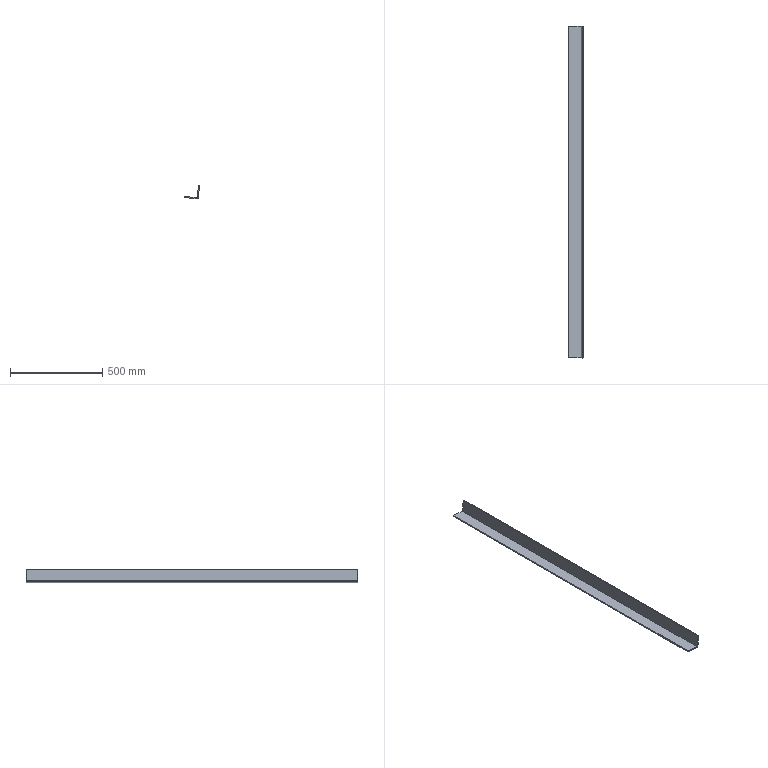Component | NX | UP_RIGHT_FRAME1800_2 | 1 solid | 8 faces | box 82.08 x 1800 x 75.23 mm | volume 1555200 mm3 | plane 8
STEP:
#1=CARTESIAN_POINT('',(0.,0.,0.));
#2=DIRECTION('',(0.,0.,1.));
#3=DIRECTION('',(1.,0.,0.));
#4=AXIS2_PLACEMENT_3D('',#1,#2,#3);
#5=CARTESIAN_POINT('',(1554.12,-7.5,442.548));
#6=VERTEX_POINT('',#5);
#7=CARTESIAN_POINT('',(1479.491,-7.5,449.997));
#8=VERTEX_POINT('',#7);
#9=CARTESIAN_POINT('',(1554.12,-7.5,442.548));
#10=DIRECTION('',(-0.9951,0.,0.09932));
#11=VECTOR('',#10,1.);
#12=LINE('',#9,#11);
#13=CARTESIAN_POINT('',(1554.12,1792.5,442.548));
#14=DIRECTION('',(0.09932,0.,0.9951));
#15=DIRECTION('',(0.9951,0.,-0.09932));
#16=AXIS2_PLACEMENT_3D('',#13,#14,#15);
#17=PLANE('',#16);
#18=CARTESIAN_POINT('',(0.,-1800.));
#19=DIRECTION('',(-1.,0.));
#20=VECTOR('',#19,1.);
#21=LINE('',#18,#20);
#22=(GEOMETRIC_REPRESENTATION_CONTEXT(2)PARAMETRIC_REPRESENTATION_CONTEXT()REPRESENTATION_CONTEXT('',''));
#23=DEFINITIONAL_REPRESENTATION('',(#21),#22);
#24=PCURVE('',#17,#23);
#25=CARTESIAN_POINT('',(1479.491,-7.5,449.997));
#26=DIRECTION('',(0.,1.,0.));
#27=DIRECTION('',(-0.9951,0.,0.09932));
#28=AXIS2_PLACEMENT_3D('',#25,#26,#27);
#29=PLANE('',#28);
#30=CARTESIAN_POINT('',(-75.,-0.));
#31=DIRECTION('',(1.,0.));
#32=VECTOR('',#31,1.);
#33=LINE('',#30,#32);
#34=(GEOMETRIC_REPRESENTATION_CONTEXT(2)PARAMETRIC_REPRESENTATION_CONTEXT()REPRESENTATION_CONTEXT('',''));
#35=DEFINITIONAL_REPRESENTATION('',(#33),#34);
#36=PCURVE('',#29,#35);
#37=SURFACE_CURVE('',#12,(#24,#36),.PCURVE_S1.);
#38=EDGE_CURVE('',#6,#8,#37,.T.);
#39=ORIENTED_EDGE('',*,*,#38,.T.);
#40=CARTESIAN_POINT('',(1479.491,1792.5,449.997));
#41=VERTEX_POINT('',#40);
#42=CARTESIAN_POINT('',(1479.491,1792.5,449.997));
#43=DIRECTION('',(0.,-1.,0.));
#44=VECTOR('',#43,1.);
#45=LINE('',#42,#44);
#46=CARTESIAN_POINT('',(-75.,0.));
#47=DIRECTION('',(0.,-1.));
#48=VECTOR('',#47,1.);
#49=LINE('',#46,#48);
#50=(GEOMETRIC_REPRESENTATION_CONTEXT(2)PARAMETRIC_REPRESENTATION_CONTEXT()REPRESENTATION_CONTEXT('',''));
#51=DEFINITIONAL_REPRESENTATION('',(#49),#50);
#52=PCURVE('',#17,#51);
#53=CARTESIAN_POINT('',(1479.491,1792.5,449.997));
#54=DIRECTION('',(0.9951,0.,-0.09932));
#55=DIRECTION('',(-0.09932,0.,-0.9951));
#56=AXIS2_PLACEMENT_3D('',#53,#54,#55);
#57=PLANE('',#56);
#58=CARTESIAN_POINT('',(0.,0.));
#59=DIRECTION('',(0.,-1.));
#60=VECTOR('',#59,1.);
#61=LINE('',#58,#60);
#62=(GEOMETRIC_REPRESENTATION_CONTEXT(2)PARAMETRIC_REPRESENTATION_CONTEXT()REPRESENTATION_CONTEXT('',''));
#63=DEFINITIONAL_REPRESENTATION('',(#61),#62);
#64=PCURVE('',#57,#63);
#65=SURFACE_CURVE('',#45,(#52,#64),.PCURVE_S1.);
#66=EDGE_CURVE('',#41,#8,#65,.T.);
#67=ORIENTED_EDGE('',*,*,#66,.F.);
#68=CARTESIAN_POINT('',(1554.12,1792.5,442.548));
#69=VERTEX_POINT('',#68);
#70=CARTESIAN_POINT('',(1554.12,1792.5,442.548));
#71=DIRECTION('',(-0.9951,0.,0.09932));
#72=VECTOR('',#71,1.);
#73=LINE('',#70,#72);
#74=CARTESIAN_POINT('',(0.,0.));
#75=DIRECTION('',(-1.,0.));
#76=VECTOR('',#75,1.);
#77=LINE('',#74,#76);
#78=(GEOMETRIC_REPRESENTATION_CONTEXT(2)PARAMETRIC_REPRESENTATION_CONTEXT()REPRESENTATION_CONTEXT('',''));
#79=DEFINITIONAL_REPRESENTATION('',(#77),#78);
#80=PCURVE('',#17,#79);
#81=CARTESIAN_POINT('',(1479.491,1792.5,449.997));
#82=DIRECTION('',(0.,1.,0.));
#83=DIRECTION('',(-0.9951,0.,0.09932));
#84=AXIS2_PLACEMENT_3D('',#81,#82,#83);
#85=PLANE('',#84);
#86=CARTESIAN_POINT('',(-75.,-0.));
#87=DIRECTION('',(1.,0.));
#88=VECTOR('',#87,1.);
#89=LINE('',#86,#88);
#90=(GEOMETRIC_REPRESENTATION_CONTEXT(2)PARAMETRIC_REPRESENTATION_CONTEXT()REPRESENTATION_CONTEXT('',''));
#91=DEFINITIONAL_REPRESENTATION('',(#89),#90);
#92=PCURVE('',#85,#91);
#93=SURFACE_CURVE('',#73,(#80,#92),.PCURVE_S1.);
#94=EDGE_CURVE('',#69,#41,#93,.T.);
#95=ORIENTED_EDGE('',*,*,#94,.F.);
#96=CARTESIAN_POINT('',(1554.12,1792.5,442.548));
#97=DIRECTION('',(0.,-1.,0.));
#98=VECTOR('',#97,1.);
#99=LINE('',#96,#98);
#100=CARTESIAN_POINT('',(0.,0.));
#101=DIRECTION('',(0.,-1.));
#102=VECTOR('',#101,1.);
#103=LINE('',#100,#102);
#104=(GEOMETRIC_REPRESENTATION_CONTEXT(2)PARAMETRIC_REPRESENTATION_CONTEXT()REPRESENTATION_CONTEXT('',''));
#105=DEFINITIONAL_REPRESENTATION('',(#103),#104);
#106=PCURVE('',#17,#105);
#107=CARTESIAN_POINT('',(1561.569,1792.5,517.177));
#108=DIRECTION('',(-0.9951,0.,0.09932));
#109=DIRECTION('',(0.09932,0.,0.9951));
#110=AXIS2_PLACEMENT_3D('',#107,#108,#109);
#111=PLANE('',#110);
#112=CARTESIAN_POINT('',(-75.,0.));
#113=DIRECTION('',(0.,-1.));
#114=VECTOR('',#113,1.);
#115=LINE('',#112,#114);
#116=(GEOMETRIC_REPRESENTATION_CONTEXT(2)PARAMETRIC_REPRESENTATION_CONTEXT()REPRESENTATION_CONTEXT('',''));
#117=DEFINITIONAL_REPRESENTATION('',(#115),#116);
#118=PCURVE('',#111,#117);
#119=SURFACE_CURVE('',#99,(#106,#118),.PCURVE_S1.);
#120=EDGE_CURVE('',#69,#6,#119,.T.);
#121=ORIENTED_EDGE('',*,*,#120,.T.);
#122=EDGE_LOOP('',(#39,#67,#95,#121));
#123=FACE_BOUND('',#122,.T.);
#124=ADVANCED_FACE('',(#123),#17,.F.);
#125=CARTESIAN_POINT('',(1480.087,-7.5,455.967));
#126=VERTEX_POINT('',#125);
#127=CARTESIAN_POINT('',(1479.491,-7.5,449.997));
#128=DIRECTION('',(0.09932,0.,0.9951));
#129=VECTOR('',#128,1.);
#130=LINE('',#127,#129);
#131=CARTESIAN_POINT('',(0.,-1800.));
#132=DIRECTION('',(-1.,0.));
#133=VECTOR('',#132,1.);
#134=LINE('',#131,#133);
#135=(GEOMETRIC_REPRESENTATION_CONTEXT(2)PARAMETRIC_REPRESENTATION_CONTEXT()REPRESENTATION_CONTEXT('',''));
#136=DEFINITIONAL_REPRESENTATION('',(#134),#135);
#137=PCURVE('',#57,#136);
#138=CARTESIAN_POINT('',(0.,0.));
#139=DIRECTION('',(0.,1.));
#140=VECTOR('',#139,1.);
#141=LINE('',#138,#140);
#142=(GEOMETRIC_REPRESENTATION_CONTEXT(2)PARAMETRIC_REPRESENTATION_CONTEXT()REPRESENTATION_CONTEXT('',''));
#143=DEFINITIONAL_REPRESENTATION('',(#141),#142);
#144=PCURVE('',#29,#143);
#145=SURFACE_CURVE('',#130,(#137,#144),.PCURVE_S1.);
#146=EDGE_CURVE('',#8,#126,#145,.T.);
#147=ORIENTED_EDGE('',*,*,#146,.T.);
#148=CARTESIAN_POINT('',(1480.087,1792.5,455.967));
#149=VERTEX_POINT('',#148);
#150=CARTESIAN_POINT('',(1480.087,1792.5,455.967));
#151=DIRECTION('',(0.,-1.,0.));
#152=VECTOR('',#151,1.);
#153=LINE('',#150,#152);
#154=CARTESIAN_POINT('',(-6.,0.));
#155=DIRECTION('',(0.,-1.));
#156=VECTOR('',#155,1.);
#157=LINE('',#154,#156);
#158=(GEOMETRIC_REPRESENTATION_CONTEXT(2)PARAMETRIC_REPRESENTATION_CONTEXT()REPRESENTATION_CONTEXT('',''));
#159=DEFINITIONAL_REPRESENTATION('',(#157),#158);
#160=PCURVE('',#57,#159);
#161=CARTESIAN_POINT('',(1480.087,1792.5,455.967));
#162=DIRECTION('',(-0.09932,0.,-0.9951));
#163=DIRECTION('',(-0.9951,0.,0.09932));
#164=AXIS2_PLACEMENT_3D('',#161,#162,#163);
#165=PLANE('',#164);
#166=CARTESIAN_POINT('',(0.,0.));
#167=DIRECTION('',(0.,-1.));
#168=VECTOR('',#167,1.);
#169=LINE('',#166,#168);
#170=(GEOMETRIC_REPRESENTATION_CONTEXT(2)PARAMETRIC_REPRESENTATION_CONTEXT()REPRESENTATION_CONTEXT('',''));
#171=DEFINITIONAL_REPRESENTATION('',(#169),#170);
#172=PCURVE('',#165,#171);
#173=SURFACE_CURVE('',#153,(#160,#172),.PCURVE_S1.);
#174=EDGE_CURVE('',#149,#126,#173,.T.);
#175=ORIENTED_EDGE('',*,*,#174,.F.);
#176=CARTESIAN_POINT('',(1479.491,1792.5,449.997));
#177=DIRECTION('',(0.09932,0.,0.9951));
#178=VECTOR('',#177,1.);
#179=LINE('',#176,#178);
#180=CARTESIAN_POINT('',(0.,0.));
#181=DIRECTION('',(-1.,0.));
#182=VECTOR('',#181,1.);
#183=LINE('',#180,#182);
#184=(GEOMETRIC_REPRESENTATION_CONTEXT(2)PARAMETRIC_REPRESENTATION_CONTEXT()REPRESENTATION_CONTEXT('',''));
#185=DEFINITIONAL_REPRESENTATION('',(#183),#184);
#186=PCURVE('',#57,#185);
#187=CARTESIAN_POINT('',(0.,0.));
#188=DIRECTION('',(0.,1.));
#189=VECTOR('',#188,1.);
#190=LINE('',#187,#189);
#191=(GEOMETRIC_REPRESENTATION_CONTEXT(2)PARAMETRIC_REPRESENTATION_CONTEXT()REPRESENTATION_CONTEXT('',''));
#192=DEFINITIONAL_REPRESENTATION('',(#190),#191);
#193=PCURVE('',#85,#192);
#194=SURFACE_CURVE('',#179,(#186,#193),.PCURVE_S1.);
#195=EDGE_CURVE('',#41,#149,#194,.T.);
#196=ORIENTED_EDGE('',*,*,#195,.F.);
#197=ORIENTED_EDGE('',*,*,#66,.T.);
#198=EDGE_LOOP('',(#147,#175,#196,#197));
#199=FACE_BOUND('',#198,.T.);
#200=ADVANCED_FACE('',(#199),#57,.F.);
#201=CARTESIAN_POINT('',(1548.746,-7.5,449.114));
#202=VERTEX_POINT('',#201);
#203=CARTESIAN_POINT('',(1480.087,-7.5,455.967));
#204=DIRECTION('',(0.9951,0.,-0.09932));
#205=VECTOR('',#204,1.);
#206=LINE('',#203,#205);
#207=CARTESIAN_POINT('',(0.,-1800.));
#208=DIRECTION('',(-1.,0.));
#209=VECTOR('',#208,1.);
#210=LINE('',#207,#209);
#211=(GEOMETRIC_REPRESENTATION_CONTEXT(2)PARAMETRIC_REPRESENTATION_CONTEXT()REPRESENTATION_CONTEXT('',''));
#212=DEFINITIONAL_REPRESENTATION('',(#210),#211);
#213=PCURVE('',#165,#212);
#214=CARTESIAN_POINT('',(0.,6.));
#215=DIRECTION('',(-1.,-0.));
#216=VECTOR('',#215,1.);
#217=LINE('',#214,#216);
#218=(GEOMETRIC_REPRESENTATION_CONTEXT(2)PARAMETRIC_REPRESENTATION_CONTEXT()REPRESENTATION_CONTEXT('',''));
#219=DEFINITIONAL_REPRESENTATION('',(#217),#218);
#220=PCURVE('',#29,#219);
#221=SURFACE_CURVE('',#206,(#213,#220),.PCURVE_S1.);
#222=EDGE_CURVE('',#126,#202,#221,.T.);
#223=ORIENTED_EDGE('',*,*,#222,.T.);
#224=CARTESIAN_POINT('',(1548.746,1792.5,449.114));
#225=VERTEX_POINT('',#224);
#226=CARTESIAN_POINT('',(1548.746,1792.5,449.114));
#227=DIRECTION('',(0.,-1.,0.));
#228=VECTOR('',#227,1.);
#229=LINE('',#226,#228);
#230=CARTESIAN_POINT('',(-69.,0.));
#231=DIRECTION('',(0.,-1.));
#232=VECTOR('',#231,1.);
#233=LINE('',#230,#232);
#234=(GEOMETRIC_REPRESENTATION_CONTEXT(2)PARAMETRIC_REPRESENTATION_CONTEXT()REPRESENTATION_CONTEXT('',''));
#235=DEFINITIONAL_REPRESENTATION('',(#233),#234);
#236=PCURVE('',#165,#235);
#237=CARTESIAN_POINT('',(1548.746,1792.5,449.114));
#238=DIRECTION('',(0.9951,0.,-0.09932));
#239=DIRECTION('',(-0.09932,0.,-0.9951));
#240=AXIS2_PLACEMENT_3D('',#237,#238,#239);
#241=PLANE('',#240);
#242=CARTESIAN_POINT('',(0.,0.));
#243=DIRECTION('',(0.,-1.));
#244=VECTOR('',#243,1.);
#245=LINE('',#242,#244);
#246=(GEOMETRIC_REPRESENTATION_CONTEXT(2)PARAMETRIC_REPRESENTATION_CONTEXT()REPRESENTATION_CONTEXT('',''));
#247=DEFINITIONAL_REPRESENTATION('',(#245),#246);
#248=PCURVE('',#241,#247);
#249=SURFACE_CURVE('',#229,(#236,#248),.PCURVE_S1.);
#250=EDGE_CURVE('',#225,#202,#249,.T.);
#251=ORIENTED_EDGE('',*,*,#250,.F.);
#252=CARTESIAN_POINT('',(1480.087,1792.5,455.967));
#253=DIRECTION('',(0.9951,0.,-0.09932));
#254=VECTOR('',#253,1.);
#255=LINE('',#252,#254);
#256=CARTESIAN_POINT('',(0.,0.));
#257=DIRECTION('',(-1.,0.));
#258=VECTOR('',#257,1.);
#259=LINE('',#256,#258);
#260=(GEOMETRIC_REPRESENTATION_CONTEXT(2)PARAMETRIC_REPRESENTATION_CONTEXT()REPRESENTATION_CONTEXT('',''));
#261=DEFINITIONAL_REPRESENTATION('',(#259),#260);
#262=PCURVE('',#165,#261);
#263=CARTESIAN_POINT('',(0.,6.));
#264=DIRECTION('',(-1.,-0.));
#265=VECTOR('',#264,1.);
#266=LINE('',#263,#265);
#267=(GEOMETRIC_REPRESENTATION_CONTEXT(2)PARAMETRIC_REPRESENTATION_CONTEXT()REPRESENTATION_CONTEXT('',''));
#268=DEFINITIONAL_REPRESENTATION('',(#266),#267);
#269=PCURVE('',#85,#268);
#270=SURFACE_CURVE('',#255,(#262,#269),.PCURVE_S1.);
#271=EDGE_CURVE('',#149,#225,#270,.T.);
#272=ORIENTED_EDGE('',*,*,#271,.F.);
#273=ORIENTED_EDGE('',*,*,#174,.T.);
#274=EDGE_LOOP('',(#223,#251,#272,#273));
#275=FACE_BOUND('',#274,.T.);
#276=ADVANCED_FACE('',(#275),#165,.F.);
#277=CARTESIAN_POINT('',(1555.599,-7.5,517.773));
#278=VERTEX_POINT('',#277);
#279=CARTESIAN_POINT('',(1548.746,-7.5,449.114));
#280=DIRECTION('',(0.09932,0.,0.9951));
#281=VECTOR('',#280,1.);
#282=LINE('',#279,#281);
#283=CARTESIAN_POINT('',(0.,-1800.));
#284=DIRECTION('',(-1.,0.));
#285=VECTOR('',#284,1.);
#286=LINE('',#283,#285);
#287=(GEOMETRIC_REPRESENTATION_CONTEXT(2)PARAMETRIC_REPRESENTATION_CONTEXT()REPRESENTATION_CONTEXT('',''));
#288=DEFINITIONAL_REPRESENTATION('',(#286),#287);
#289=PCURVE('',#241,#288);
#290=CARTESIAN_POINT('',(-69.,6.));
#291=DIRECTION('',(0.,1.));
#292=VECTOR('',#291,1.);
#293=LINE('',#290,#292);
#294=(GEOMETRIC_REPRESENTATION_CONTEXT(2)PARAMETRIC_REPRESENTATION_CONTEXT()REPRESENTATION_CONTEXT('',''));
#295=DEFINITIONAL_REPRESENTATION('',(#293),#294);
#296=PCURVE('',#29,#295);
#297=SURFACE_CURVE('',#282,(#289,#296),.PCURVE_S1.);
#298=EDGE_CURVE('',#202,#278,#297,.T.);
#299=ORIENTED_EDGE('',*,*,#298,.T.);
#300=CARTESIAN_POINT('',(1555.599,1792.5,517.773));
#301=VERTEX_POINT('',#300);
#302=CARTESIAN_POINT('',(1555.599,1792.5,517.773));
#303=DIRECTION('',(0.,-1.,0.));
#304=VECTOR('',#303,1.);
#305=LINE('',#302,#304);
#306=CARTESIAN_POINT('',(-69.,0.));
#307=DIRECTION('',(0.,-1.));
#308=VECTOR('',#307,1.);
#309=LINE('',#306,#308);
#310=(GEOMETRIC_REPRESENTATION_CONTEXT(2)PARAMETRIC_REPRESENTATION_CONTEXT()REPRESENTATION_CONTEXT('',''));
#311=DEFINITIONAL_REPRESENTATION('',(#309),#310);
#312=PCURVE('',#241,#311);
#313=CARTESIAN_POINT('',(1555.599,1792.5,517.773));
#314=DIRECTION('',(-0.09932,0.,-0.9951));
#315=DIRECTION('',(-0.9951,0.,0.09932));
#316=AXIS2_PLACEMENT_3D('',#313,#314,#315);
#317=PLANE('',#316);
#318=CARTESIAN_POINT('',(0.,0.));
#319=DIRECTION('',(0.,-1.));
#320=VECTOR('',#319,1.);
#321=LINE('',#318,#320);
#322=(GEOMETRIC_REPRESENTATION_CONTEXT(2)PARAMETRIC_REPRESENTATION_CONTEXT()REPRESENTATION_CONTEXT('',''));
#323=DEFINITIONAL_REPRESENTATION('',(#321),#322);
#324=PCURVE('',#317,#323);
#325=SURFACE_CURVE('',#305,(#312,#324),.PCURVE_S1.);
#326=EDGE_CURVE('',#301,#278,#325,.T.);
#327=ORIENTED_EDGE('',*,*,#326,.F.);
#328=CARTESIAN_POINT('',(1548.746,1792.5,449.114));
#329=DIRECTION('',(0.09932,0.,0.9951));
#330=VECTOR('',#329,1.);
#331=LINE('',#328,#330);
#332=CARTESIAN_POINT('',(0.,0.));
#333=DIRECTION('',(-1.,0.));
#334=VECTOR('',#333,1.);
#335=LINE('',#332,#334);
#336=(GEOMETRIC_REPRESENTATION_CONTEXT(2)PARAMETRIC_REPRESENTATION_CONTEXT()REPRESENTATION_CONTEXT('',''));
#337=DEFINITIONAL_REPRESENTATION('',(#335),#336);
#338=PCURVE('',#241,#337);
#339=CARTESIAN_POINT('',(-69.,6.));
#340=DIRECTION('',(0.,1.));
#341=VECTOR('',#340,1.);
#342=LINE('',#339,#341);
#343=(GEOMETRIC_REPRESENTATION_CONTEXT(2)PARAMETRIC_REPRESENTATION_CONTEXT()REPRESENTATION_CONTEXT('',''));
#344=DEFINITIONAL_REPRESENTATION('',(#342),#343);
#345=PCURVE('',#85,#344);
#346=SURFACE_CURVE('',#331,(#338,#345),.PCURVE_S1.);
#347=EDGE_CURVE('',#225,#301,#346,.T.);
#348=ORIENTED_EDGE('',*,*,#347,.F.);
#349=ORIENTED_EDGE('',*,*,#250,.T.);
#350=EDGE_LOOP('',(#299,#327,#348,#349));
#351=FACE_BOUND('',#350,.T.);
#352=ADVANCED_FACE('',(#351),#241,.F.);
#353=CARTESIAN_POINT('',(1561.569,-7.5,517.177));
#354=VERTEX_POINT('',#353);
#355=CARTESIAN_POINT('',(1555.599,-7.5,517.773));
#356=DIRECTION('',(0.9951,0.,-0.09932));
#357=VECTOR('',#356,1.);
#358=LINE('',#355,#357);
#359=CARTESIAN_POINT('',(0.,-1800.));
#360=DIRECTION('',(-1.,0.));
#361=VECTOR('',#360,1.);
#362=LINE('',#359,#361);
#363=(GEOMETRIC_REPRESENTATION_CONTEXT(2)PARAMETRIC_REPRESENTATION_CONTEXT()REPRESENTATION_CONTEXT('',''));
#364=DEFINITIONAL_REPRESENTATION('',(#362),#363);
#365=PCURVE('',#317,#364);
#366=CARTESIAN_POINT('',(-69.,75.));
#367=DIRECTION('',(-1.,0.));
#368=VECTOR('',#367,1.);
#369=LINE('',#366,#368);
#370=(GEOMETRIC_REPRESENTATION_CONTEXT(2)PARAMETRIC_REPRESENTATION_CONTEXT()REPRESENTATION_CONTEXT('',''));
#371=DEFINITIONAL_REPRESENTATION('',(#369),#370);
#372=PCURVE('',#29,#371);
#373=SURFACE_CURVE('',#358,(#365,#372),.PCURVE_S1.);
#374=EDGE_CURVE('',#278,#354,#373,.T.);
#375=ORIENTED_EDGE('',*,*,#374,.T.);
#376=CARTESIAN_POINT('',(1561.569,1792.5,517.177));
#377=VERTEX_POINT('',#376);
#378=CARTESIAN_POINT('',(1561.569,1792.5,517.177));
#379=DIRECTION('',(0.,-1.,0.));
#380=VECTOR('',#379,1.);
#381=LINE('',#378,#380);
#382=CARTESIAN_POINT('',(-6.,0.));
#383=DIRECTION('',(0.,-1.));
#384=VECTOR('',#383,1.);
#385=LINE('',#382,#384);
#386=(GEOMETRIC_REPRESENTATION_CONTEXT(2)PARAMETRIC_REPRESENTATION_CONTEXT()REPRESENTATION_CONTEXT('',''));
#387=DEFINITIONAL_REPRESENTATION('',(#385),#386);
#388=PCURVE('',#317,#387);
#389=CARTESIAN_POINT('',(0.,0.));
#390=DIRECTION('',(0.,-1.));
#391=VECTOR('',#390,1.);
#392=LINE('',#389,#391);
#393=(GEOMETRIC_REPRESENTATION_CONTEXT(2)PARAMETRIC_REPRESENTATION_CONTEXT()REPRESENTATION_CONTEXT('',''));
#394=DEFINITIONAL_REPRESENTATION('',(#392),#393);
#395=PCURVE('',#111,#394);
#396=SURFACE_CURVE('',#381,(#388,#395),.PCURVE_S1.);
#397=EDGE_CURVE('',#377,#354,#396,.T.);
#398=ORIENTED_EDGE('',*,*,#397,.F.);
#399=CARTESIAN_POINT('',(1555.599,1792.5,517.773));
#400=DIRECTION('',(0.9951,0.,-0.09932));
#401=VECTOR('',#400,1.);
#402=LINE('',#399,#401);
#403=CARTESIAN_POINT('',(0.,0.));
#404=DIRECTION('',(-1.,0.));
#405=VECTOR('',#404,1.);
#406=LINE('',#403,#405);
#407=(GEOMETRIC_REPRESENTATION_CONTEXT(2)PARAMETRIC_REPRESENTATION_CONTEXT()REPRESENTATION_CONTEXT('',''));
#408=DEFINITIONAL_REPRESENTATION('',(#406),#407);
#409=PCURVE('',#317,#408);
#410=CARTESIAN_POINT('',(-69.,75.));
#411=DIRECTION('',(-1.,0.));
#412=VECTOR('',#411,1.);
#413=LINE('',#410,#412);
#414=(GEOMETRIC_REPRESENTATION_CONTEXT(2)PARAMETRIC_REPRESENTATION_CONTEXT()REPRESENTATION_CONTEXT('',''));
#415=DEFINITIONAL_REPRESENTATION('',(#413),#414);
#416=PCURVE('',#85,#415);
#417=SURFACE_CURVE('',#402,(#409,#416),.PCURVE_S1.);
#418=EDGE_CURVE('',#301,#377,#417,.T.);
#419=ORIENTED_EDGE('',*,*,#418,.F.);
#420=ORIENTED_EDGE('',*,*,#326,.T.);
#421=EDGE_LOOP('',(#375,#398,#419,#420));
#422=FACE_BOUND('',#421,.T.);
#423=ADVANCED_FACE('',(#422),#317,.F.);
#424=CARTESIAN_POINT('',(1561.569,-7.5,517.177));
#425=DIRECTION('',(-0.09932,0.,-0.9951));
#426=VECTOR('',#425,1.);
#427=LINE('',#424,#426);
#428=CARTESIAN_POINT('',(0.,-1800.));
#429=DIRECTION('',(-1.,0.));
#430=VECTOR('',#429,1.);
#431=LINE('',#428,#430);
#432=(GEOMETRIC_REPRESENTATION_CONTEXT(2)PARAMETRIC_REPRESENTATION_CONTEXT()REPRESENTATION_CONTEXT('',''));
#433=DEFINITIONAL_REPRESENTATION('',(#431),#432);
#434=PCURVE('',#111,#433);
#435=CARTESIAN_POINT('',(-75.,75.));
#436=DIRECTION('',(0.,-1.));
#437=VECTOR('',#436,1.);
#438=LINE('',#435,#437);
#439=(GEOMETRIC_REPRESENTATION_CONTEXT(2)PARAMETRIC_REPRESENTATION_CONTEXT()REPRESENTATION_CONTEXT('',''));
#440=DEFINITIONAL_REPRESENTATION('',(#438),#439);
#441=PCURVE('',#29,#440);
#442=SURFACE_CURVE('',#427,(#434,#441),.PCURVE_S1.);
#443=EDGE_CURVE('',#354,#6,#442,.T.);
#444=ORIENTED_EDGE('',*,*,#443,.T.);
#445=ORIENTED_EDGE('',*,*,#120,.F.);
#446=CARTESIAN_POINT('',(1561.569,1792.5,517.177));
#447=DIRECTION('',(-0.09932,0.,-0.9951));
#448=VECTOR('',#447,1.);
#449=LINE('',#446,#448);
#450=CARTESIAN_POINT('',(0.,0.));
#451=DIRECTION('',(-1.,0.));
#452=VECTOR('',#451,1.);
#453=LINE('',#450,#452);
#454=(GEOMETRIC_REPRESENTATION_CONTEXT(2)PARAMETRIC_REPRESENTATION_CONTEXT()REPRESENTATION_CONTEXT('',''));
#455=DEFINITIONAL_REPRESENTATION('',(#453),#454);
#456=PCURVE('',#111,#455);
#457=CARTESIAN_POINT('',(-75.,75.));
#458=DIRECTION('',(0.,-1.));
#459=VECTOR('',#458,1.);
#460=LINE('',#457,#459);
#461=(GEOMETRIC_REPRESENTATION_CONTEXT(2)PARAMETRIC_REPRESENTATION_CONTEXT()REPRESENTATION_CONTEXT('',''));
#462=DEFINITIONAL_REPRESENTATION('',(#460),#461);
#463=PCURVE('',#85,#462);
#464=SURFACE_CURVE('',#449,(#456,#463),.PCURVE_S1.);
#465=EDGE_CURVE('',#377,#69,#464,.T.);
#466=ORIENTED_EDGE('',*,*,#465,.F.);
#467=ORIENTED_EDGE('',*,*,#397,.T.);
#468=EDGE_LOOP('',(#444,#445,#466,#467));
#469=FACE_BOUND('',#468,.T.);
#470=ADVANCED_FACE('',(#469),#111,.F.);
#471=ORIENTED_EDGE('',*,*,#94,.T.);
#472=ORIENTED_EDGE('',*,*,#195,.T.);
#473=ORIENTED_EDGE('',*,*,#271,.T.);
#474=ORIENTED_EDGE('',*,*,#347,.T.);
#475=ORIENTED_EDGE('',*,*,#418,.T.);
#476=ORIENTED_EDGE('',*,*,#465,.T.);
#477=EDGE_LOOP('',(#471,#472,#473,#474,#475,#476));
#478=FACE_BOUND('',#477,.T.);
#479=ADVANCED_FACE('',(#478),#85,.T.);
#480=ORIENTED_EDGE('',*,*,#38,.F.);
#481=ORIENTED_EDGE('',*,*,#443,.F.);
#482=ORIENTED_EDGE('',*,*,#374,.F.);
#483=ORIENTED_EDGE('',*,*,#298,.F.);
#484=ORIENTED_EDGE('',*,*,#222,.F.);
#485=ORIENTED_EDGE('',*,*,#146,.F.);
#486=EDGE_LOOP('',(#480,#481,#482,#483,#484,#485));
#487=FACE_BOUND('',#486,.T.);
#488=ADVANCED_FACE('',(#487),#29,.F.);
#489=CLOSED_SHELL('',(#124,#200,#276,#352,#423,#470,#479,#488));
#490=MANIFOLD_SOLID_BREP('',#489);
#491=(LENGTH_UNIT()NAMED_UNIT(*)SI_UNIT(.MILLI.,.METRE.));
#492=UNCERTAINTY_MEASURE_WITH_UNIT(LENGTH_MEASURE(0.0000001),#491,'','');
#493=(NAMED_UNIT(*)PLANE_ANGLE_UNIT()SI_UNIT($,.RADIAN.));
#494=(NAMED_UNIT(*)SI_UNIT($,.STERADIAN.)SOLID_ANGLE_UNIT());
#495=(GEOMETRIC_REPRESENTATION_CONTEXT(3)GLOBAL_UNCERTAINTY_ASSIGNED_CONTEXT((#492))GLOBAL_UNIT_ASSIGNED_CONTEXT((#491,#493,#494))REPRESENTATION_CONTEXT('',''));
#496=ADVANCED_BREP_SHAPE_REPRESENTATION('',(#4,#490),#495);